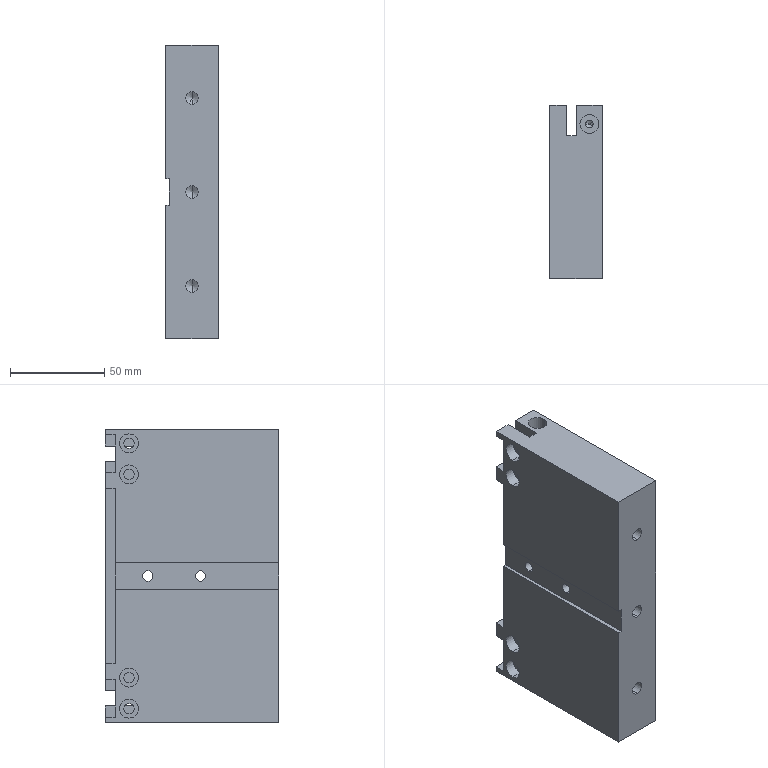Component | SolidWorks | PointedHeadBaseA-1 | 1 solid | 113 faces | box 28 x 92 x 156 mm | volume 367359 mm3 | cylinder 50 | plane 40 | cone 23 | commonest cylinder face diameters 10 x16 5.5 x12 4.2 x12 6.8 x6 3.3 x4
build123d program:
from build123d import *

# Parameters (mm, degrees)
SKETCH1_W                                            = 28
SKETCH1_H                                            = 156
EXTRUDE1_DEPTH                                       = 92
SKETCH2_W                                            = 5.2
SKETCH2_H                                            = 156
CUT_EXTRUDE1_DEPTH                                   = 5.2
SKETCH3_W                                            = 9
SKETCH3_H                                            = 20
CUT_EXTRUDE2_DEPTH                                   = 5.2
SKETCH4_W                                            = 9
SKETCH4_H                                            = 93
CUT_EXTRUDE3_DEPTH                                   = 5.2
SKETCH7_W                                            = 5.2
SKETCH7_H                                            = 156
CUT_EXTRUDE5_DEPTH                                   = 11
SKETCH5_W                                            = 13.8
SKETCH5_H                                            = 8
CUT_EXTRUDE4_DEPTH                                   = 16.2
SKETCH8_R                                            = 5
CUT_EXTRUDE6_DEPTH                                   = 13.2
M5_TAPPED_HOLE1_D                                    = 4.2
M5_TAPPED_HOLE1_DEPTH                                = 12
M5_TAPPED_HOLE1_TIP                                  = 1.262
CUT_EXTRUDE7_START                                   = -13.2
SKETCH11_R                                           = 5
CUT_EXTRUDE7_DEPTH                                   = 13.2
M5_TAPPED_HOLE2_D                                    = 4.2
M5_TAPPED_HOLE2_DEPTH                                = 14
M5_TAPPED_HOLE2_TIP                                  = 1.262
SKETCH16_R                                           = 2.75
CUT_EXTRUDE10_DEPTH                                  = 12
SKETCH17_R                                           = 5
CUT_EXTRUDE11_DEPTH                                  = 5.5
M5_TAPPED_HOLE3_D                                    = 4.2
M5_TAPPED_HOLE3_DEPTH                                = 14
M5_TAPPED_HOLE3_TIP                                  = 1.262
M8_TAPPED_HOLE1_D                                    = 6.8
M8_TAPPED_HOLE1_DEPTH                                = 22.25
M8_TAPPED_HOLE1_TIP                                  = 2.043
SKETCH22_W                                           = 14
SKETCH22_H                                           = 86.8
CUT_EXTRUDE12_DEPTH                                  = 2
COUNTERBORE_FOR_M5_SOCKET_HEAD_CAP_SCREW_D           = 5.5
COUNTERBORE_FOR_M5_SOCKET_HEAD_CAP_SCREW_CBORE_D     = 10
COUNTERBORE_FOR_M5_SOCKET_HEAD_CAP_SCREW_CBORE_DEPTH = 5
M4_TAPPED_HOLE1_D                                    = 3.3
M4_TAPPED_HOLE1_DEPTH                                = 11.5
M4_TAPPED_HOLE1_TIP                                  = 0.9914


with BuildPart() as part:
    # Sketch1 → Extrude1 (new body)
    with BuildSketch(Plane(origin=(0, 0, 0), x_dir=(1, 0, 0), z_dir=(0, 1, 0))):
        with Locations((14, -78)):
            Rectangle(SKETCH1_W, SKETCH1_H)
    extrude(amount=EXTRUDE1_DEPTH)

    # Sketch2 → Cut-Extrude1 (cut)
    with BuildSketch(Plane(origin=(0, 92, 0), x_dir=(1, 0, 0), z_dir=(0, 1, 0))):
        with Locations((11.6, -78)):
            Rectangle(SKETCH2_W, SKETCH2_H)
    extrude(amount=-CUT_EXTRUDE1_DEPTH, mode=Mode.SUBTRACT)

    # Sketch3 → Cut-Extrude2 (cut)
    with BuildSketch(Plane(origin=(0, 92, 0), x_dir=(1, 0, 0), z_dir=(0, 1, 0))):
        with Locations((4.5, -143)):
            Rectangle(SKETCH3_W, SKETCH3_H)
        with Locations((4.5, -13)):
            Rectangle(SKETCH3_W, SKETCH3_H)
    extrude(amount=-CUT_EXTRUDE2_DEPTH, mode=Mode.SUBTRACT)

    # Sketch4 → Cut-Extrude3 (cut)
    with BuildSketch(Plane(origin=(0, 92, 0), x_dir=(1, 0, 0), z_dir=(0, 1, 0))):
        with Locations((4.5, -78)):
            Rectangle(SKETCH4_W, SKETCH4_H)
    extrude(amount=-CUT_EXTRUDE3_DEPTH, mode=Mode.SUBTRACT)

    # Sketch7 → Cut-Extrude5 (cut)
    with BuildSketch(Plane(origin=(0, 86.8, 0), x_dir=(1, 0, 0), z_dir=(0, 1, 0))):
        with Locations((11.6, -78)):
            Rectangle(SKETCH7_W, SKETCH7_H)
    extrude(amount=-CUT_EXTRUDE5_DEPTH, mode=Mode.SUBTRACT)

    # Sketch5 → Cut-Extrude4 (cut)
    with BuildSketch(Plane(origin=(0, 92, 0), x_dir=(1, 0, 0), z_dir=(0, 1, 0))):
        with Locations((21.1, -143)):
            Rectangle(SKETCH5_W, SKETCH5_H)
        with Locations((21.1, -13)):
            Rectangle(SKETCH5_W, SKETCH5_H)
    extrude(amount=-CUT_EXTRUDE4_DEPTH, mode=Mode.SUBTRACT)

    # Sketch8 → Cut-Extrude6 (cut)
    with BuildSketch(Plane.XY.offset(156)):
        with Locations((21.1, 82)):
            Circle(SKETCH8_R)
    extrude(amount=-CUT_EXTRUDE6_DEPTH, mode=Mode.SUBTRACT)

    # M5 Tapped Hole1
    with Locations(Plane.XY.offset(139)):
        with Locations((21.1, 82)):
            Hole(M5_TAPPED_HOLE1_D / 2, depth=M5_TAPPED_HOLE1_DEPTH)
            with Locations((0, 0, -(M5_TAPPED_HOLE1_DEPTH + M5_TAPPED_HOLE1_TIP / 2))):  # 118° drill point
                Cone(0, M5_TAPPED_HOLE1_D / 2, M5_TAPPED_HOLE1_TIP, mode=Mode.SUBTRACT)

    # Sketch11 → Cut-Extrude7 (cut)
    with BuildSketch(Plane(origin=(0, 0, 0), x_dir=(-1, 0, 0), z_dir=(0, 0, -1)).offset(CUT_EXTRUDE7_START)):
        with Locations(Location((-21.1, 82, 0), (0, 0, 180))):
            Circle(SKETCH11_R)
    extrude(amount=CUT_EXTRUDE7_DEPTH, mode=Mode.SUBTRACT)

    # M5 Tapped Hole2
    with Locations(Plane(origin=(0, 0, 17), x_dir=(-1, 0, 0), z_dir=(0, 0, -1))):
        with Locations((-21.1, 82)):
            Hole(M5_TAPPED_HOLE2_D / 2, depth=M5_TAPPED_HOLE2_DEPTH)
            with Locations((0, 0, -(M5_TAPPED_HOLE2_DEPTH + M5_TAPPED_HOLE2_TIP / 2))):  # 118° drill point
                Cone(0, M5_TAPPED_HOLE2_D / 2, M5_TAPPED_HOLE2_TIP, mode=Mode.SUBTRACT)

    # Sketch16 → Cut-Extrude10 (cut)
    with BuildSketch(Plane.ZY):
        with Locations((132, 79.5)):
            Circle(SKETCH16_R)
        with Locations((148.5, 79.5)):
            Circle(SKETCH16_R)
        with Locations((24, 79.5)):
            Circle(SKETCH16_R)
        with Locations((7.5, 79.5)):
            Circle(SKETCH16_R)
    extrude(amount=-CUT_EXTRUDE10_DEPTH, mode=Mode.SUBTRACT)

    # Sketch17 → Cut-Extrude11 (cut)
    with BuildSketch(Plane.ZY):
        with Locations((132, 79.5)):
            Circle(SKETCH17_R)
        with Locations((148.5, 79.5)):
            Circle(SKETCH17_R)
        with Locations((7.5, 79.5)):
            Circle(SKETCH17_R)
        with Locations((24, 79.5)):
            Circle(SKETCH17_R)
    extrude(amount=-CUT_EXTRUDE11_DEPTH, mode=Mode.SUBTRACT)

    # M5 Tapped Hole3
    with Locations(Plane(origin=(0, 92, 0), x_dir=(-1, 0, 0), z_dir=(0, 1, 0))):
        with Locations((-21.1, 123), (-21.1, 93), (-21.1, 63), (-21.1, 33)):
            Hole(M5_TAPPED_HOLE3_D / 2, depth=M5_TAPPED_HOLE3_DEPTH)
            with Locations((0, 0, -(M5_TAPPED_HOLE3_DEPTH + M5_TAPPED_HOLE3_TIP / 2))):  # 118° drill point
                Cone(0, M5_TAPPED_HOLE3_D / 2, M5_TAPPED_HOLE3_TIP, mode=Mode.SUBTRACT)

    # M8 Tapped Hole1
    with Locations(Plane.XZ):
        with Locations((14, 78), (14, 28), (14, 128)):
            Hole(M8_TAPPED_HOLE1_D / 2, depth=M8_TAPPED_HOLE1_DEPTH)
            with Locations((0, 0, -(M8_TAPPED_HOLE1_DEPTH + M8_TAPPED_HOLE1_TIP / 2))):  # 118° drill point
                Cone(0, M8_TAPPED_HOLE1_D / 2, M8_TAPPED_HOLE1_TIP, mode=Mode.SUBTRACT)

    # Sketch22 → Cut-Extrude12 (cut)
    with BuildSketch(Plane.ZY):
        with Locations((78, 43.4)):
            Rectangle(SKETCH22_W, SKETCH22_H)
    extrude(amount=-CUT_EXTRUDE12_DEPTH, mode=Mode.SUBTRACT)

    # Counterbore for M5 Socket Head Cap Screw (through all)
    with Locations(Plane(origin=(28, 0, 0), x_dir=(0, 0, -1), z_dir=(1, 0, 0))):
        with Locations((-78, 41.5), (-78, 69.5)):
            CounterBoreHole(COUNTERBORE_FOR_M5_SOCKET_HEAD_CAP_SCREW_D / 2, COUNTERBORE_FOR_M5_SOCKET_HEAD_CAP_SCREW_CBORE_D / 2, COUNTERBORE_FOR_M5_SOCKET_HEAD_CAP_SCREW_CBORE_DEPTH)

    # M4 Tapped Hole1
    with Locations(Plane(origin=(28, 0, 0), x_dir=(0, 0, -1), z_dir=(1, 0, 0))):
        with Locations((-110, 72), (-46, 72)):
            Hole(M4_TAPPED_HOLE1_D / 2, depth=M4_TAPPED_HOLE1_DEPTH)
            with Locations((0, 0, -(M4_TAPPED_HOLE1_DEPTH + M4_TAPPED_HOLE1_TIP / 2))):  # 118° drill point
                Cone(0, M4_TAPPED_HOLE1_D / 2, M4_TAPPED_HOLE1_TIP, mode=Mode.SUBTRACT)


solid = part.part

# Placed as in the assembly
solid = solid.moved(Location((10.917, -9.628, -195.387), (0, 0, 0)))